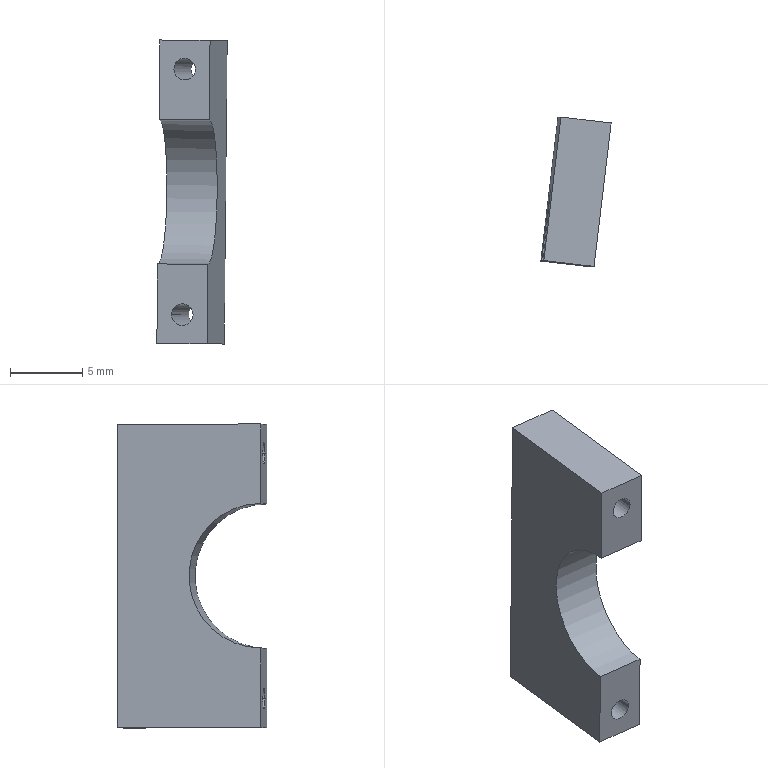Component | SolidWorks | Card-1 | 1 solid | 12 faces | box 4.86 x 10.34 x 21.04 mm | volume 562 mm3 | plane 7 | cylinder 5 | commonest cylinder face diameters 1.5 x4 10 x1 | material 45
build123d program:
from build123d import *

# Parameters (mm, degrees)
SKETCH2_W           = 3.5
SKETCH2_H           = 10
BOSS_EXTRUDE1_DEPTH = 10.5
SKETCH3_R           = 0.75
CUT_EXTRUDE1_DEPTH  = 15.916
SKETCH4_R           = 5
CUT_EXTRUDE2_DEPTH  = 18.073


with BuildPart() as part:
    # Sketch2 → Boss-Extrude1 (new, symmetric)
    with BuildSketch(Plane(origin=(0, 0, 0), x_dir=(1, 0, 0), z_dir=(0, 1, 0))):
        with Locations((-1.75, 8)):
            Rectangle(SKETCH2_W, SKETCH2_H)
    extrude(amount=BOSS_EXTRUDE1_DEPTH, both=True)

    # Sketch3 → Cut-Extrude1 (cut, through all)
    with BuildSketch(Plane(origin=(0, 0, -13), x_dir=(-1, 0, 0), z_dir=(0, 0, -1))):
        with Locations((1.75, -8.5)):
            Circle(SKETCH3_R)
        with Locations(Location((1.75, 8.5, 0), (0, 0, 180))):
            Circle(SKETCH3_R)
    extrude(amount=-CUT_EXTRUDE1_DEPTH, mode=Mode.SUBTRACT)

    # Sketch4 → Cut-Extrude2 (cut, through all)
    with BuildSketch(Plane.ZY.offset(3.5)):
        with Locations((-3, 0)):
            Circle(SKETCH4_R)
    extrude(amount=-CUT_EXTRUDE2_DEPTH, mode=Mode.SUBTRACT)


solid = part.part

# Placed as in the assembly
solid = solid.moved(Location((3.695, 63.752, -1.882), (89.933, -6.795, 179.435)))
STEP:
#1=COLOUR_RGB('',0.7922,0.8196,0.9333);
#2=FILL_AREA_STYLE_COLOUR('',#1);
#3=FILL_AREA_STYLE('',(#2));
#4=SURFACE_STYLE_FILL_AREA(#3);
#5=SURFACE_SIDE_STYLE('',(#4));
#6=SURFACE_STYLE_USAGE(.BOTH.,#5);
#7=PRESENTATION_STYLE_ASSIGNMENT((#6));
#8=CARTESIAN_POINT('',(0.1953,2.623,-0.4092));
#9=VERTEX_POINT('',#8);
#10=CARTESIAN_POINT('',(0.2539,2.616,-0.4098));
#11=VERTEX_POINT('',#10);
#12=CARTESIAN_POINT('',(0.2246,2.619,-0.4095));
#13=DIRECTION('',(0.1183,0.993,-0.001159));
#14=DIRECTION('',(-0.9929,0.1183,0.009724));
#15=AXIS2_PLACEMENT_3D('',#12,#13,#14);
#16=CIRCLE('',#15,0.02953);
#17=EDGE_CURVE('',#9,#11,#16,.T.);
#18=ORIENTED_EDGE('',*,*,#17,.F.);
#19=CARTESIAN_POINT('',(0.2419,3.013,-0.4097));
#20=VERTEX_POINT('',#19);
#21=CARTESIAN_POINT('',(0.1953,2.623,-0.4092));
#22=DIRECTION('',(0.1183,0.993,-0.001159));
#23=VECTOR('',#22,39.37);
#24=LINE('',#21,#23);
#25=EDGE_CURVE('',#9,#20,#24,.T.);
#26=ORIENTED_EDGE('',*,*,#25,.T.);
#27=CARTESIAN_POINT('',(0.3005,3.006,-0.4103));
#28=VERTEX_POINT('',#27);
#29=CARTESIAN_POINT('',(0.2712,3.01,-0.41));
#30=DIRECTION('',(0.1183,0.993,-0.001159));
#31=DIRECTION('',(-0.9929,0.1183,0.009724));
#32=AXIS2_PLACEMENT_3D('',#29,#30,#31);
#33=CIRCLE('',#32,0.02953);
#34=EDGE_CURVE('',#20,#28,#33,.T.);
#35=ORIENTED_EDGE('',*,*,#34,.T.);
#36=CARTESIAN_POINT('',(0.2539,2.616,-0.4098));
#37=DIRECTION('',(0.1183,0.993,-0.001159));
#38=VECTOR('',#37,39.37);
#39=LINE('',#36,#38);
#40=EDGE_CURVE('',#11,#28,#39,.T.);
#41=ORIENTED_EDGE('',*,*,#40,.F.);
#42=EDGE_LOOP('',(#18,#26,#35,#41));
#43=FACE_OUTER_BOUND('',#42,.T.);
#44=CARTESIAN_POINT('',(0.2246,2.619,-0.4095));
#45=DIRECTION('',(0.1183,0.993,-0.001159));
#46=DIRECTION('',(0.9929,-0.1183,-0.009724));
#47=AXIS2_PLACEMENT_3D('',#44,#45,#46);
#48=CYLINDRICAL_SURFACE('',#47,0.02953);
#49=ADVANCED_FACE('',(#43),#48,.F.);
#50=CARTESIAN_POINT('',(0.2018,2.623,0.26));
#51=VERTEX_POINT('',#50);
#52=CARTESIAN_POINT('',(0.2605,2.616,0.2594));
#53=VERTEX_POINT('',#52);
#54=CARTESIAN_POINT('',(0.2311,2.619,0.2597));
#55=DIRECTION('',(0.1183,0.993,-0.001159));
#56=DIRECTION('',(0.9929,-0.1183,-0.009724));
#57=AXIS2_PLACEMENT_3D('',#54,#55,#56);
#58=CIRCLE('',#57,0.02953);
#59=EDGE_CURVE('',#51,#53,#58,.T.);
#60=ORIENTED_EDGE('',*,*,#59,.F.);
#61=CARTESIAN_POINT('',(0.2484,3.013,0.2596));
#62=VERTEX_POINT('',#61);
#63=CARTESIAN_POINT('',(0.2018,2.623,0.26));
#64=DIRECTION('',(0.1183,0.993,-0.001159));
#65=VECTOR('',#64,39.37);
#66=LINE('',#63,#65);
#67=EDGE_CURVE('',#51,#62,#66,.T.);
#68=ORIENTED_EDGE('',*,*,#67,.T.);
#69=CARTESIAN_POINT('',(0.307,3.006,0.259));
#70=VERTEX_POINT('',#69);
#71=CARTESIAN_POINT('',(0.2777,3.01,0.2593));
#72=DIRECTION('',(0.1183,0.993,-0.001159));
#73=DIRECTION('',(0.9929,-0.1183,-0.009724));
#74=AXIS2_PLACEMENT_3D('',#71,#72,#73);
#75=CIRCLE('',#74,0.02953);
#76=EDGE_CURVE('',#62,#70,#75,.T.);
#77=ORIENTED_EDGE('',*,*,#76,.T.);
#78=CARTESIAN_POINT('',(0.2605,2.616,0.2594));
#79=DIRECTION('',(0.1183,0.993,-0.001159));
#80=VECTOR('',#79,39.37);
#81=LINE('',#78,#80);
#82=EDGE_CURVE('',#53,#70,#81,.T.);
#83=ORIENTED_EDGE('',*,*,#82,.F.);
#84=EDGE_LOOP('',(#60,#68,#77,#83));
#85=FACE_OUTER_BOUND('',#84,.T.);
#86=CARTESIAN_POINT('',(0.2311,2.619,0.2597));
#87=DIRECTION('',(0.1183,0.993,-0.001159));
#88=DIRECTION('',(0.9929,-0.1183,-0.009724));
#89=AXIS2_PLACEMENT_3D('',#86,#87,#88);
#90=CYLINDRICAL_SURFACE('',#89,0.02953);
#91=ADVANCED_FACE('',(#85),#90,.F.);
#92=CARTESIAN_POINT('',(0.2311,2.619,0.2597));
#93=DIRECTION('',(0.1183,0.993,-0.001159));
#94=DIRECTION('',(0.9929,-0.1183,-0.009724));
#95=AXIS2_PLACEMENT_3D('',#92,#93,#94);
#96=CIRCLE('',#95,0.02953);
#97=EDGE_CURVE('',#53,#51,#96,.T.);
#98=ORIENTED_EDGE('',*,*,#97,.T.);
#99=ORIENTED_EDGE('',*,*,#59,.T.);
#100=EDGE_LOOP('',(#98,#99));
#101=FACE_BOUND('',#100,.T.);
#102=CARTESIAN_POINT('',(0.1614,2.627,0.1226));
#103=VERTEX_POINT('',#102);
#104=CARTESIAN_POINT('',(0.1635,2.627,0.3391));
#105=VERTEX_POINT('',#104);
#106=CARTESIAN_POINT('',(0.1554,2.627,-0.4876));
#107=DIRECTION('',(0.009793,0.,1.));
#108=VECTOR('',#107,39.37);
#109=LINE('',#106,#108);
#110=EDGE_CURVE('',#103,#105,#109,.T.);
#111=ORIENTED_EDGE('',*,*,#110,.F.);
#112=CARTESIAN_POINT('',(0.2982,2.611,0.1213));
#113=VERTEX_POINT('',#112);
#114=CARTESIAN_POINT('',(0.1614,2.627,0.1226));
#115=DIRECTION('',(0.9929,-0.1183,-0.009724));
#116=VECTOR('',#115,39.37);
#117=LINE('',#114,#116);
#118=EDGE_CURVE('',#103,#113,#117,.T.);
#119=ORIENTED_EDGE('',*,*,#118,.T.);
#120=CARTESIAN_POINT('',(0.3003,2.611,0.3378));
#121=VERTEX_POINT('',#120);
#122=CARTESIAN_POINT('',(0.2922,2.611,-0.4889));
#123=DIRECTION('',(0.009793,0.,1.));
#124=VECTOR('',#123,39.37);
#125=LINE('',#122,#124);
#126=EDGE_CURVE('',#113,#121,#125,.T.);
#127=ORIENTED_EDGE('',*,*,#126,.T.);
#128=CARTESIAN_POINT('',(0.1635,2.627,0.3391));
#129=DIRECTION('',(-0.9929,0.1183,0.009724));
#130=VECTOR('',#129,39.37);
#131=LINE('',#128,#130);
#132=EDGE_CURVE('',#121,#105,#131,.T.);
#133=ORIENTED_EDGE('',*,*,#132,.T.);
#134=EDGE_LOOP('',(#111,#119,#127,#133));
#135=FACE_OUTER_BOUND('',#134,.T.);
#136=CARTESIAN_POINT('',(0.1554,2.627,-0.4876));
#137=DIRECTION('',(0.1183,0.993,-0.001159));
#138=DIRECTION('',(0.9929,-0.1183,-0.009724));
#139=AXIS2_PLACEMENT_3D('',#136,#137,#138);
#140=PLANE('',#139);
#141=ADVANCED_FACE('',(#101,#135),#140,.F.);
#142=CARTESIAN_POINT('',(0.1554,2.627,-0.4876));
#143=VERTEX_POINT('',#142);
#144=CARTESIAN_POINT('',(0.1575,2.627,-0.2711));
#145=VERTEX_POINT('',#144);
#146=CARTESIAN_POINT('',(0.1554,2.627,-0.4876));
#147=DIRECTION('',(0.009793,0.,1.));
#148=VECTOR('',#147,39.37);
#149=LINE('',#146,#148);
#150=EDGE_CURVE('',#143,#145,#149,.T.);
#151=ORIENTED_EDGE('',*,*,#150,.T.);
#152=CARTESIAN_POINT('',(0.1595,2.627,-0.07424));
#153=DIRECTION('',(0.9929,-0.1183,-0.009724));
#154=DIRECTION('',(-0.1183,-0.993,0.001159));
#155=AXIS2_PLACEMENT_3D('',#152,#153,#154);
#156=CIRCLE('',#155,0.1969);
#157=EDGE_CURVE('',#145,#103,#156,.T.);
#158=ORIENTED_EDGE('',*,*,#157,.T.);
#159=ORIENTED_EDGE('',*,*,#110,.T.);
#160=CARTESIAN_POINT('',(0.2101,3.018,0.3387));
#161=VERTEX_POINT('',#160);
#162=CARTESIAN_POINT('',(0.1635,2.627,0.3391));
#163=DIRECTION('',(0.1183,0.993,-0.001159));
#164=VECTOR('',#163,39.37);
#165=LINE('',#162,#164);
#166=EDGE_CURVE('',#105,#161,#165,.T.);
#167=ORIENTED_EDGE('',*,*,#166,.T.);
#168=CARTESIAN_POINT('',(0.202,3.018,-0.4881));
#169=VERTEX_POINT('',#168);
#170=CARTESIAN_POINT('',(0.202,3.018,-0.4881));
#171=DIRECTION('',(0.009793,0.,1.));
#172=VECTOR('',#171,39.37);
#173=LINE('',#170,#172);
#174=EDGE_CURVE('',#169,#161,#173,.T.);
#175=ORIENTED_EDGE('',*,*,#174,.F.);
#176=CARTESIAN_POINT('',(0.1554,2.627,-0.4876));
#177=DIRECTION('',(0.1183,0.993,-0.001159));
#178=VECTOR('',#177,39.37);
#179=LINE('',#176,#178);
#180=EDGE_CURVE('',#143,#169,#179,.T.);
#181=ORIENTED_EDGE('',*,*,#180,.F.);
#182=EDGE_LOOP('',(#151,#158,#159,#167,#175,#181));
#183=FACE_OUTER_BOUND('',#182,.T.);
#184=CARTESIAN_POINT('',(0.1554,2.627,-0.4876));
#185=DIRECTION('',(0.9929,-0.1183,-0.009724));
#186=DIRECTION('',(-0.1183,-0.993,0.001159));
#187=AXIS2_PLACEMENT_3D('',#184,#185,#186);
#188=PLANE('',#187);
#189=ADVANCED_FACE('',(#183),#188,.F.);
#190=CARTESIAN_POINT('',(0.2712,3.01,-0.41));
#191=DIRECTION('',(0.1183,0.993,-0.001159));
#192=DIRECTION('',(-0.9929,0.1183,0.009724));
#193=AXIS2_PLACEMENT_3D('',#190,#191,#192);
#194=CIRCLE('',#193,0.02953);
#195=EDGE_CURVE('',#28,#20,#194,.T.);
#196=ORIENTED_EDGE('',*,*,#195,.F.);
#197=ORIENTED_EDGE('',*,*,#34,.F.);
#198=EDGE_LOOP('',(#196,#197));
#199=FACE_BOUND('',#198,.T.);
#200=CARTESIAN_POINT('',(0.2777,3.01,0.2593));
#201=DIRECTION('',(0.1183,0.993,-0.001159));
#202=DIRECTION('',(0.9929,-0.1183,-0.009724));
#203=AXIS2_PLACEMENT_3D('',#200,#201,#202);
#204=CIRCLE('',#203,0.02953);
#205=EDGE_CURVE('',#70,#62,#204,.T.);
#206=ORIENTED_EDGE('',*,*,#205,.F.);
#207=ORIENTED_EDGE('',*,*,#76,.F.);
#208=EDGE_LOOP('',(#206,#207));
#209=FACE_BOUND('',#208,.T.);
#210=CARTESIAN_POINT('',(0.3469,3.002,0.3373));
#211=VERTEX_POINT('',#210);
#212=CARTESIAN_POINT('',(0.2101,3.018,0.3387));
#213=DIRECTION('',(0.9929,-0.1183,-0.009724));
#214=VECTOR('',#213,39.37);
#215=LINE('',#212,#214);
#216=EDGE_CURVE('',#161,#211,#215,.T.);
#217=ORIENTED_EDGE('',*,*,#216,.T.);
#218=CARTESIAN_POINT('',(0.3388,3.002,-0.4894));
#219=VERTEX_POINT('',#218);
#220=CARTESIAN_POINT('',(0.3388,3.002,-0.4894));
#221=DIRECTION('',(0.009793,0.,1.));
#222=VECTOR('',#221,39.37);
#223=LINE('',#220,#222);
#224=EDGE_CURVE('',#219,#211,#223,.T.);
#225=ORIENTED_EDGE('',*,*,#224,.F.);
#226=CARTESIAN_POINT('',(0.202,3.018,-0.4881));
#227=DIRECTION('',(0.9929,-0.1183,-0.009724));
#228=VECTOR('',#227,39.37);
#229=LINE('',#226,#228);
#230=EDGE_CURVE('',#169,#219,#229,.T.);
#231=ORIENTED_EDGE('',*,*,#230,.F.);
#232=ORIENTED_EDGE('',*,*,#174,.T.);
#233=EDGE_LOOP('',(#217,#225,#231,#232));
#234=FACE_OUTER_BOUND('',#233,.T.);
#235=CARTESIAN_POINT('',(0.202,3.018,-0.4881));
#236=DIRECTION('',(-0.1183,-0.993,0.001159));
#237=DIRECTION('',(-0.9929,0.1183,0.009724));
#238=AXIS2_PLACEMENT_3D('',#235,#236,#237);
#239=PLANE('',#238);
#240=ADVANCED_FACE('',(#199,#209,#234),#239,.F.);
#241=ORIENTED_EDGE('',*,*,#126,.F.);
#242=CARTESIAN_POINT('',(0.2943,2.611,-0.2724));
#243=VERTEX_POINT('',#242);
#244=CARTESIAN_POINT('',(0.2963,2.611,-0.07558));
#245=DIRECTION('',(0.9929,-0.1183,-0.009724));
#246=DIRECTION('',(-0.1183,-0.993,0.001159));
#247=AXIS2_PLACEMENT_3D('',#244,#245,#246);
#248=CIRCLE('',#247,0.1969);
#249=EDGE_CURVE('',#243,#113,#248,.T.);
#250=ORIENTED_EDGE('',*,*,#249,.F.);
#251=CARTESIAN_POINT('',(0.2922,2.611,-0.4889));
#252=VERTEX_POINT('',#251);
#253=CARTESIAN_POINT('',(0.2922,2.611,-0.4889));
#254=DIRECTION('',(0.009793,0.,1.));
#255=VECTOR('',#254,39.37);
#256=LINE('',#253,#255);
#257=EDGE_CURVE('',#252,#243,#256,.T.);
#258=ORIENTED_EDGE('',*,*,#257,.F.);
#259=CARTESIAN_POINT('',(0.2922,2.611,-0.4889));
#260=DIRECTION('',(-0.1183,-0.993,0.001159));
#261=VECTOR('',#260,39.37);
#262=LINE('',#259,#261);
#263=EDGE_CURVE('',#219,#252,#262,.T.);
#264=ORIENTED_EDGE('',*,*,#263,.F.);
#265=ORIENTED_EDGE('',*,*,#224,.T.);
#266=CARTESIAN_POINT('',(0.3003,2.611,0.3378));
#267=DIRECTION('',(-0.1183,-0.993,0.001159));
#268=VECTOR('',#267,39.37);
#269=LINE('',#266,#268);
#270=EDGE_CURVE('',#211,#121,#269,.T.);
#271=ORIENTED_EDGE('',*,*,#270,.T.);
#272=EDGE_LOOP('',(#241,#250,#258,#264,#265,#271));
#273=FACE_OUTER_BOUND('',#272,.T.);
#274=CARTESIAN_POINT('',(0.2922,2.611,-0.4889));
#275=DIRECTION('',(-0.9929,0.1183,0.009724));
#276=DIRECTION('',(0.1183,0.993,-0.001159));
#277=AXIS2_PLACEMENT_3D('',#274,#275,#276);
#278=PLANE('',#277);
#279=ADVANCED_FACE('',(#273),#278,.F.);
#280=CARTESIAN_POINT('',(0.2246,2.619,-0.4095));
#281=DIRECTION('',(0.1183,0.993,-0.001159));
#282=DIRECTION('',(-0.9929,0.1183,0.009724));
#283=AXIS2_PLACEMENT_3D('',#280,#281,#282);
#284=CIRCLE('',#283,0.02953);
#285=EDGE_CURVE('',#11,#9,#284,.T.);
#286=ORIENTED_EDGE('',*,*,#285,.T.);
#287=ORIENTED_EDGE('',*,*,#17,.T.);
#288=EDGE_LOOP('',(#286,#287));
#289=FACE_BOUND('',#288,.T.);
#290=ORIENTED_EDGE('',*,*,#257,.T.);
#291=CARTESIAN_POINT('',(0.1575,2.627,-0.2711));
#292=DIRECTION('',(-0.9929,0.1183,0.009724));
#293=VECTOR('',#292,39.37);
#294=LINE('',#291,#293);
#295=EDGE_CURVE('',#243,#145,#294,.T.);
#296=ORIENTED_EDGE('',*,*,#295,.T.);
#297=ORIENTED_EDGE('',*,*,#150,.F.);
#298=CARTESIAN_POINT('',(0.1554,2.627,-0.4876));
#299=DIRECTION('',(-0.9929,0.1183,0.009724));
#300=VECTOR('',#299,39.37);
#301=LINE('',#298,#300);
#302=EDGE_CURVE('',#252,#143,#301,.T.);
#303=ORIENTED_EDGE('',*,*,#302,.F.);
#304=EDGE_LOOP('',(#290,#296,#297,#303));
#305=FACE_OUTER_BOUND('',#304,.T.);
#306=CARTESIAN_POINT('',(0.1554,2.627,-0.4876));
#307=DIRECTION('',(0.1183,0.993,-0.001159));
#308=DIRECTION('',(0.9929,-0.1183,-0.009724));
#309=AXIS2_PLACEMENT_3D('',#306,#307,#308);
#310=PLANE('',#309);
#311=ADVANCED_FACE('',(#289,#305),#310,.F.);
#312=ORIENTED_EDGE('',*,*,#180,.T.);
#313=ORIENTED_EDGE('',*,*,#230,.T.);
#314=ORIENTED_EDGE('',*,*,#263,.T.);
#315=ORIENTED_EDGE('',*,*,#302,.T.);
#316=EDGE_LOOP('',(#312,#313,#314,#315));
#317=FACE_OUTER_BOUND('',#316,.T.);
#318=CARTESIAN_POINT('',(0.1414,2.51,-0.4875));
#319=DIRECTION('',(-0.009793,-0.,-1.));
#320=DIRECTION('',(-0.1183,-0.993,0.001159));
#321=AXIS2_PLACEMENT_3D('',#318,#319,#320);
#322=PLANE('',#321);
#323=ADVANCED_FACE('',(#317),#322,.T.);
#324=ORIENTED_EDGE('',*,*,#166,.F.);
#325=ORIENTED_EDGE('',*,*,#132,.F.);
#326=ORIENTED_EDGE('',*,*,#270,.F.);
#327=ORIENTED_EDGE('',*,*,#216,.F.);
#328=EDGE_LOOP('',(#324,#325,#326,#327));
#329=FACE_OUTER_BOUND('',#328,.T.);
#330=CARTESIAN_POINT('',(0.1495,2.51,0.3393));
#331=DIRECTION('',(-0.009793,-0.,-1.));
#332=DIRECTION('',(-0.1183,-0.993,0.001159));
#333=AXIS2_PLACEMENT_3D('',#330,#331,#332);
#334=PLANE('',#333);
#335=ADVANCED_FACE('',(#329),#334,.F.);
#336=ORIENTED_EDGE('',*,*,#67,.F.);
#337=ORIENTED_EDGE('',*,*,#97,.F.);
#338=ORIENTED_EDGE('',*,*,#82,.T.);
#339=ORIENTED_EDGE('',*,*,#205,.T.);
#340=EDGE_LOOP('',(#336,#337,#338,#339));
#341=FACE_OUTER_BOUND('',#340,.T.);
#342=CARTESIAN_POINT('',(0.2311,2.619,0.2597));
#343=DIRECTION('',(0.1183,0.993,-0.001159));
#344=DIRECTION('',(0.9929,-0.1183,-0.009724));
#345=AXIS2_PLACEMENT_3D('',#342,#343,#344);
#346=CYLINDRICAL_SURFACE('',#345,0.02953);
#347=ADVANCED_FACE('',(#341),#346,.F.);
#348=ORIENTED_EDGE('',*,*,#25,.F.);
#349=ORIENTED_EDGE('',*,*,#285,.F.);
#350=ORIENTED_EDGE('',*,*,#40,.T.);
#351=ORIENTED_EDGE('',*,*,#195,.T.);
#352=EDGE_LOOP('',(#348,#349,#350,#351));
#353=FACE_OUTER_BOUND('',#352,.T.);
#354=CARTESIAN_POINT('',(0.2246,2.619,-0.4095));
#355=DIRECTION('',(0.1183,0.993,-0.001159));
#356=DIRECTION('',(0.9929,-0.1183,-0.009724));
#357=AXIS2_PLACEMENT_3D('',#354,#355,#356);
#358=CYLINDRICAL_SURFACE('',#357,0.02953);
#359=ADVANCED_FACE('',(#353),#358,.F.);
#360=ORIENTED_EDGE('',*,*,#157,.F.);
#361=ORIENTED_EDGE('',*,*,#295,.F.);
#362=ORIENTED_EDGE('',*,*,#249,.T.);
#363=ORIENTED_EDGE('',*,*,#118,.F.);
#364=EDGE_LOOP('',(#360,#361,#362,#363));
#365=FACE_OUTER_BOUND('',#364,.T.);
#366=CARTESIAN_POINT('',(0.1595,2.627,-0.07424));
#367=DIRECTION('',(0.9929,-0.1183,-0.009724));
#368=DIRECTION('',(-0.1183,-0.993,0.001159));
#369=AXIS2_PLACEMENT_3D('',#366,#367,#368);
#370=CYLINDRICAL_SURFACE('',#369,0.1969);
#371=ADVANCED_FACE('',(#365),#370,.F.);
#372=CLOSED_SHELL('',(#49,#91,#141,#189,#240,#279,#311,#323,#335,#347,#359,#371));
#373=MANIFOLD_SOLID_BREP('',#372);
#374=STYLED_ITEM('',(#7),#373);
#375=PRESENTATION_LAYER_ASSIGNMENT('','',(#374));
#376=CARTESIAN_POINT('',(0.,0.,0.));
#377=DIRECTION('',(0.,0.,1.));
#378=DIRECTION('',(1.,0.,0.));
#379=AXIS2_PLACEMENT_3D('',#376,#377,#378);
#380=(LENGTH_UNIT()NAMED_UNIT(*)SI_UNIT($,.METRE.));
#381=LENGTH_MEASURE_WITH_UNIT(LENGTH_MEASURE(0.0254),#380);
#382=DIMENSIONAL_EXPONENTS(1.,0.,0.,0.,0.,0.,0.);
#383=(CONVERSION_BASED_UNIT('',#381)LENGTH_UNIT()NAMED_UNIT(#382));
#384=UNCERTAINTY_MEASURE_WITH_UNIT(LENGTH_MEASURE(0.00001),#383,'','');
#385=(NAMED_UNIT(*)PLANE_ANGLE_UNIT()SI_UNIT($,.RADIAN.));
#386=(NAMED_UNIT(*)SI_UNIT($,.STERADIAN.)SOLID_ANGLE_UNIT());
#387=(GEOMETRIC_REPRESENTATION_CONTEXT(3)GLOBAL_UNCERTAINTY_ASSIGNED_CONTEXT((#384))GLOBAL_UNIT_ASSIGNED_CONTEXT((#383,#385,#386))REPRESENTATION_CONTEXT('',''));
#388=ADVANCED_BREP_SHAPE_REPRESENTATION('',(#373,#379),#387);
#389=(LENGTH_UNIT()NAMED_UNIT(*)SI_UNIT($,.METRE.));
#390=LENGTH_MEASURE_WITH_UNIT(LENGTH_MEASURE(0.0254),#389);
#391=DIMENSIONAL_EXPONENTS(1.,0.,0.,0.,0.,0.,0.);
#392=(CONVERSION_BASED_UNIT('',#390)LENGTH_UNIT()NAMED_UNIT(#391));
#393=UNCERTAINTY_MEASURE_WITH_UNIT(LENGTH_MEASURE(0.00001),#392,'','');
#394=(NAMED_UNIT(*)PLANE_ANGLE_UNIT()SI_UNIT($,.RADIAN.));
#395=(NAMED_UNIT(*)SI_UNIT($,.STERADIAN.)SOLID_ANGLE_UNIT());
#396=(GEOMETRIC_REPRESENTATION_CONTEXT(3)GLOBAL_UNCERTAINTY_ASSIGNED_CONTEXT((#393))GLOBAL_UNIT_ASSIGNED_CONTEXT((#392,#394,#395))REPRESENTATION_CONTEXT('',''));
#397=MECHANICAL_DESIGN_GEOMETRIC_PRESENTATION_REPRESENTATION('',(#374),#396);